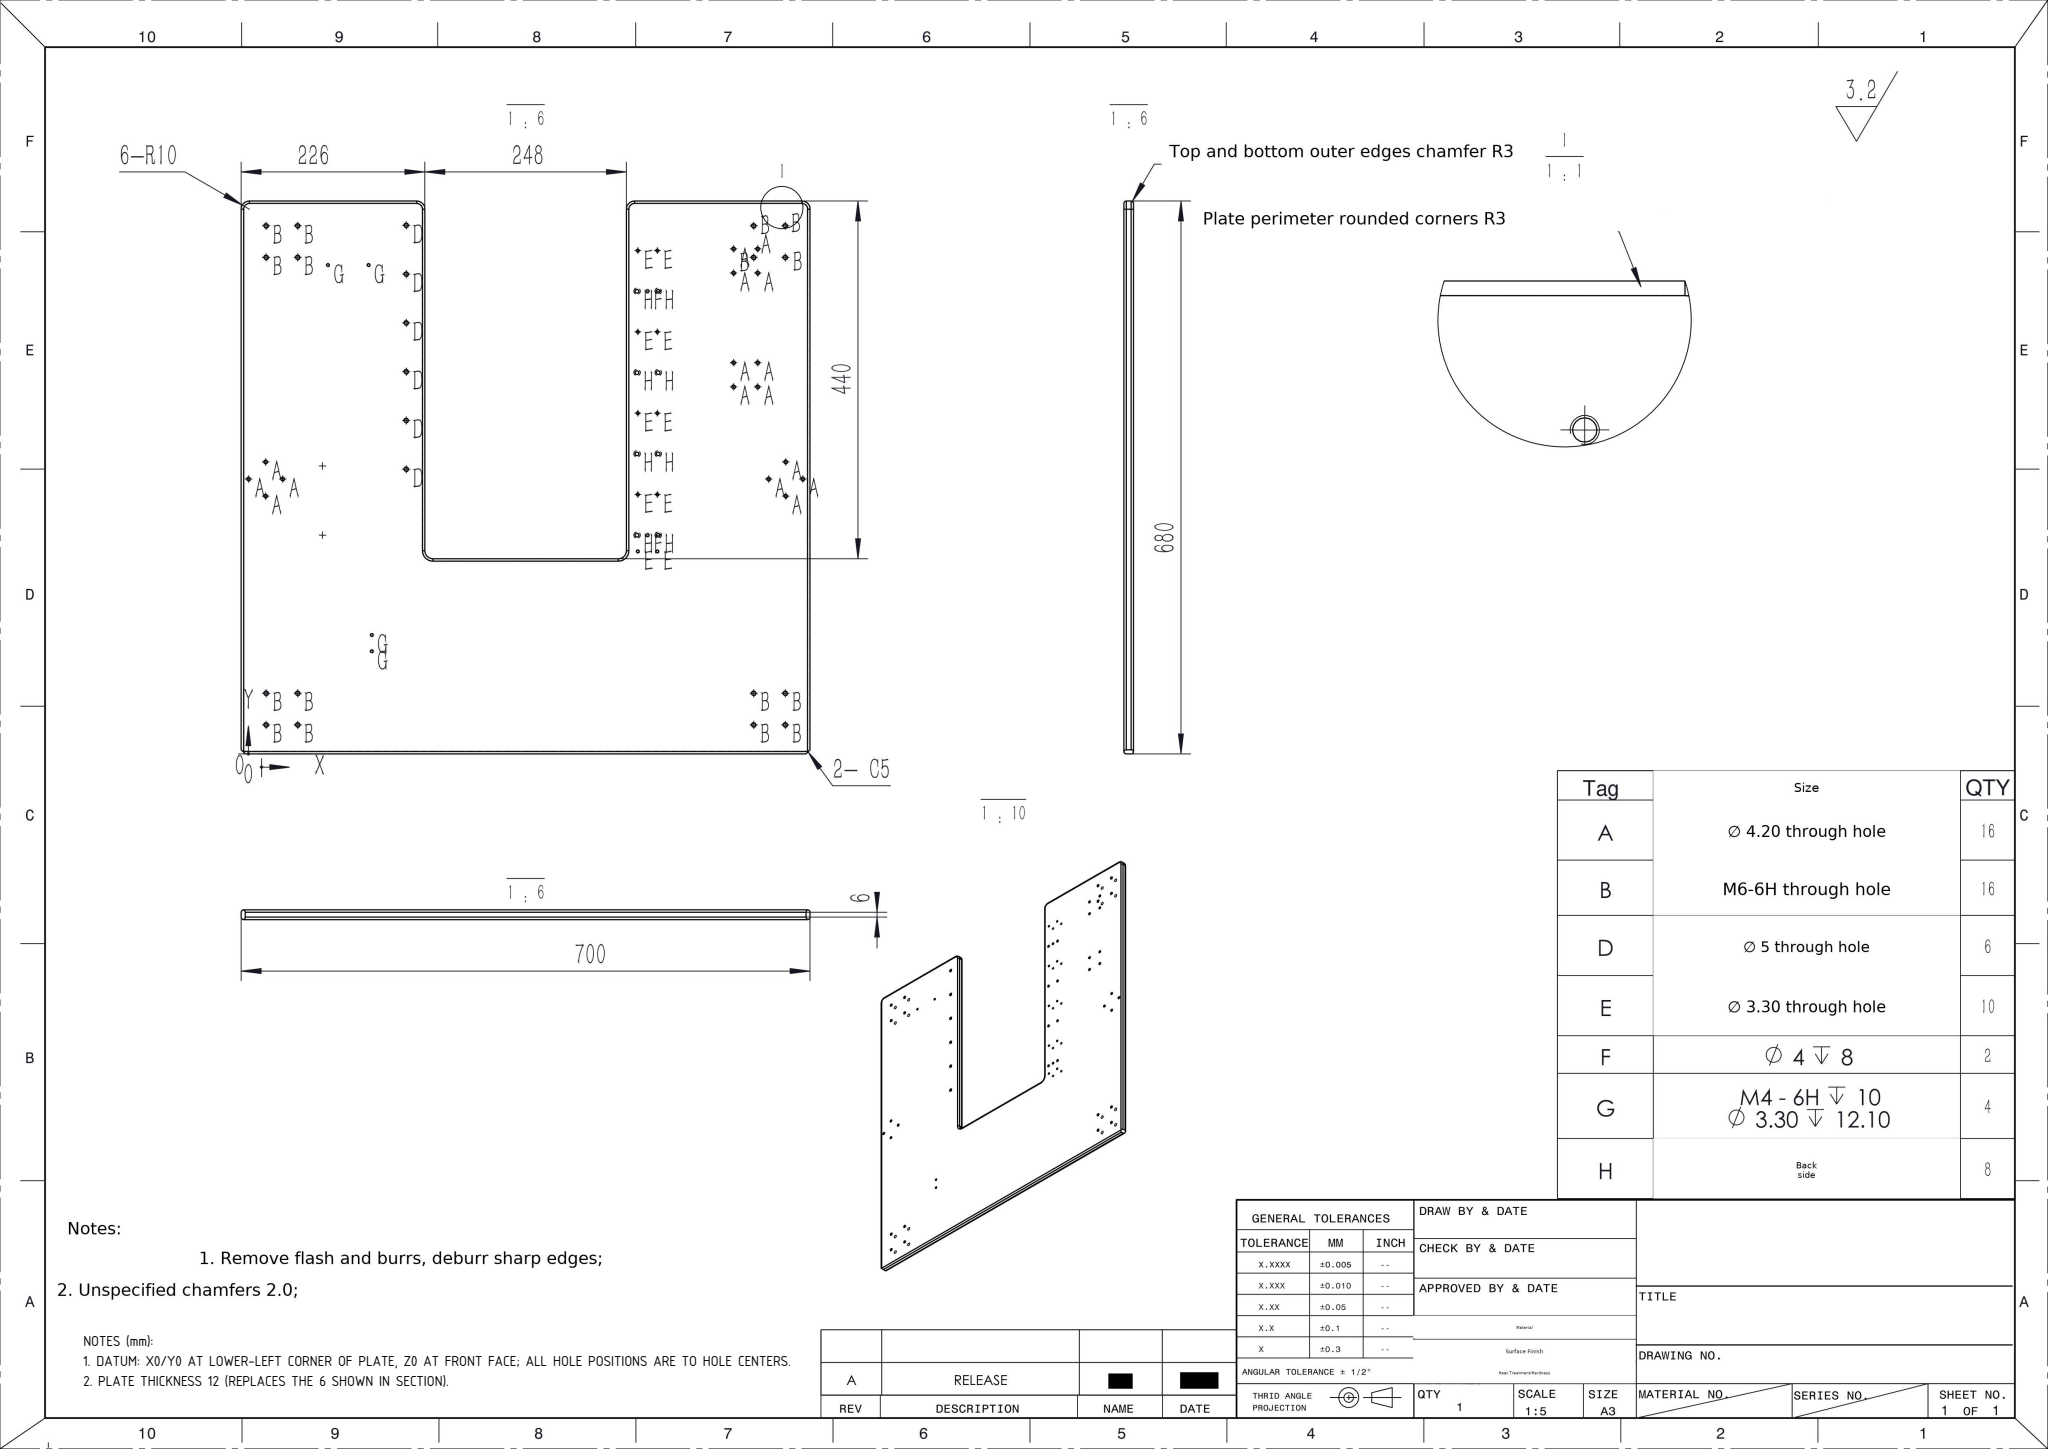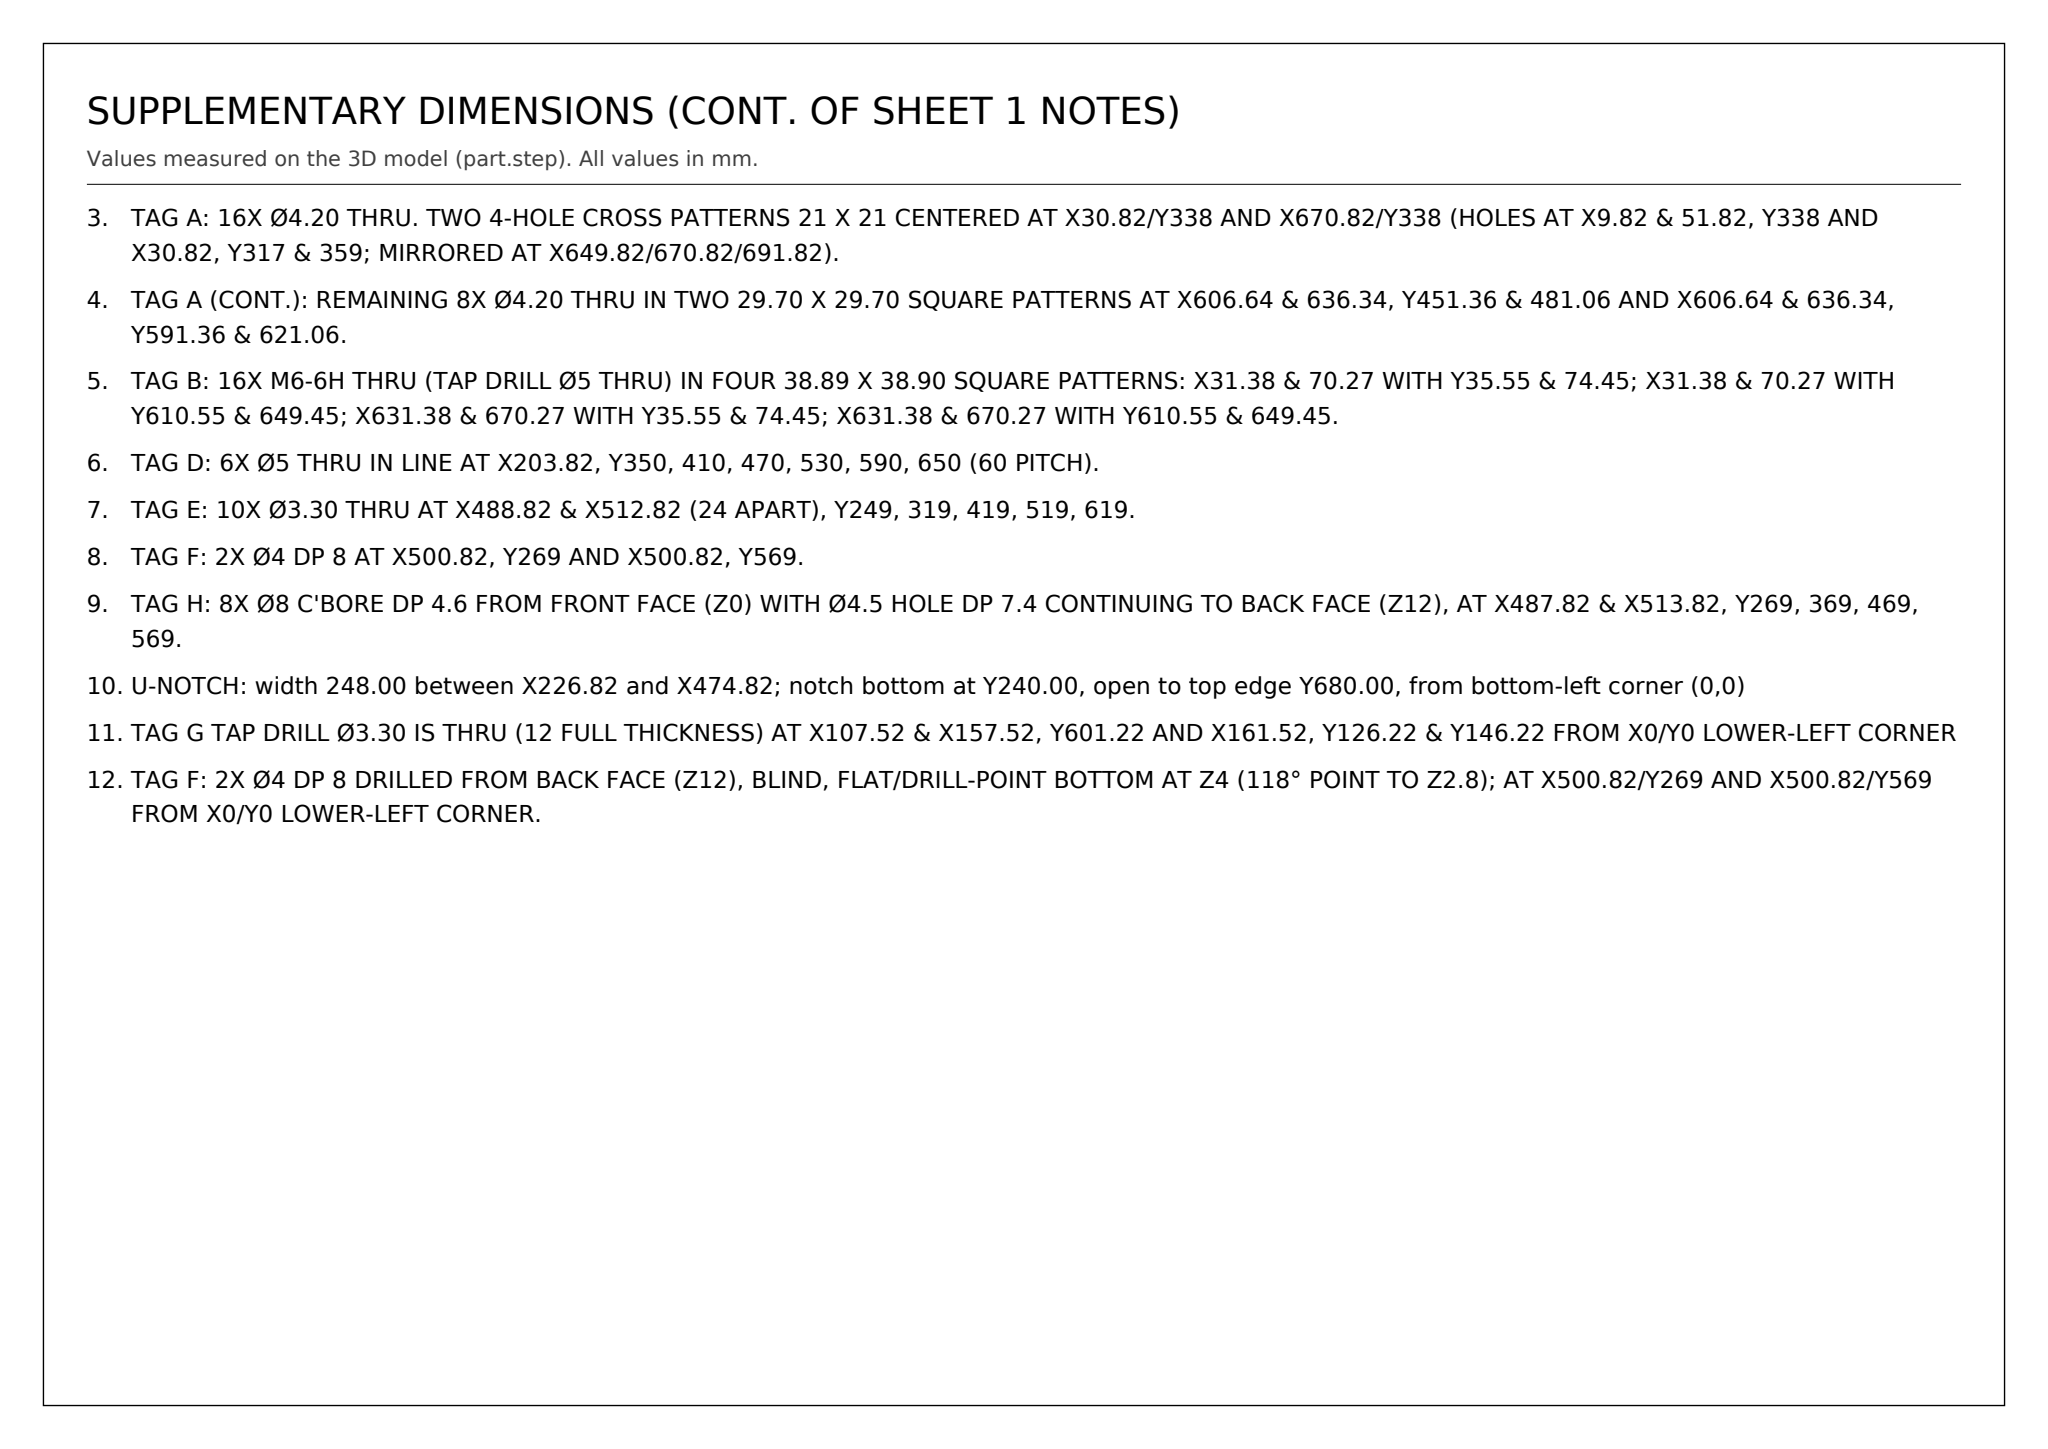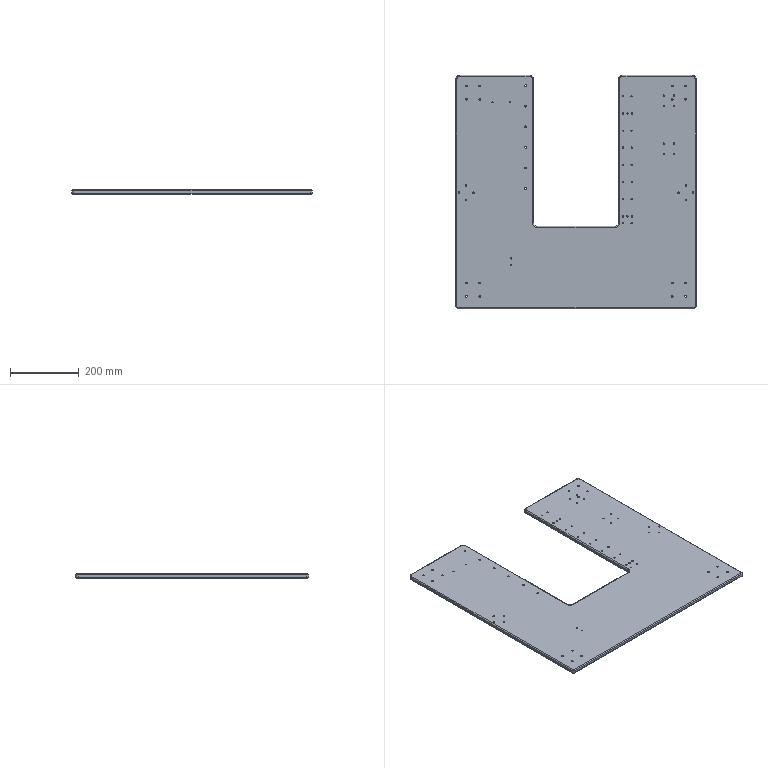Part | SolidWorks | mm | 1 solid | 198 faces | box 700 x 680 x 12 mm | volume 4375576 mm3 | cylinder 162 | plane 20 | torus 12 | cone 4 | commonest cylinder face diameters 5 x44 4.2 x32 3.3 x28 8 x16 4.5 x16 6 x16 20 x6 4 x4
Drawing notes:
DATUM: X0/Y0 AT LOWER-LEFT CORNER OF PLATE, Z0 AT FRONT FACE; ALL HOLE POSITIONS ARE TO HOLE CENTERS. | from the solid: origin_note: positions from min corner of bbox 701.648 x 680.824 x 12.0
PLATE THICKNESS 12 (REPLACES THE 6 SHOWN IN SECTION). | from the solid: bbox_xyz z = 12.0; all THRU cylinders length 12.0
TAG A: 16X Ø4.20 THRU. TWO 4-HOLE CROSS PATTERNS 21 X 21 CENTERED AT X30.82/Y338 AND X670.82/Y338 (HOLES AT X9.82 & 51.82, Y338 AND X30.82, Y317 & 359; MIRRORED AT X649.82/670.82/691.82). | from the solid: cylinders dia 4.2 z at (9.82,338),(30.82,317),(30.82,359),(51.82,338),(649.82,338),(670.82,317),(670.82,359),(691.82,338), length 12.0
TAG A (CONT.): REMAINING 8X Ø4.20 THRU IN TWO 29.70 X 29.70 SQUARE PATTERNS AT X606.64 & 636.34, Y451.36 & 481.06 AND X606.64 & 636.34, Y591.36 & 621.06. | from the solid: cylinders dia 4.2 z at (606.64/636.34, 451.36/481.06) and (606.64/636.34, 591.36/621.06), length 12.0
TAG B: 16X M6-6H THRU (TAP DRILL Ø5 THRU) IN FOUR 38.89 X 38.90 SQUARE PATTERNS: X31.38 & 70.27 WITH Y35.55 & 74.45; X31.38 & 70.27 WITH Y610.55 & 649.45; X631.38 & 670.27 WITH Y35.55 & 74.45; X631.38 & 670.27 WITH Y610.55 & 649.45. | from the solid: cylinders dia 5.0 z at x 31.38/70.27/631.38/670.27 with y 35.55/74.45/610.55/649.45, length 12.0
TAG D: 6X Ø5 THRU IN LINE AT X203.82, Y350, 410, 470, 530, 590, 650 (60 PITCH). | from the solid: cylinders dia 5.0 z at (203.82, 350/410/470/530/590/650), length 12.0
TAG E: 10X Ø3.30 THRU AT X488.82 & X512.82 (24 APART), Y249, 319, 419, 519, 619. | from the solid: cylinders dia 3.3 z at (488.82 and 512.82, y 249/319/419/519/619), length 12.0
TAG F: 2X Ø4 DP 8 AT X500.82, Y269 AND X500.82, Y569. | from the solid: cylinders dia 4.0 z at (500.82,269) and (500.82,569), length 8.0
TAG H: 8X Ø8 C'BORE DP 4.6 FROM FRONT FACE (Z0) WITH Ø4.5 HOLE DP 7.4 CONTINUING TO BACK FACE (Z12), AT X487.82 & X513.82, Y269, 369, 469, 569. | from the solid: Flat c'bore bottoms at z=4.6 over X483.8-491.8 and X509.8-517.8 with Y265-273/365-373/465-473/565-573 (8 places, 8x8 => Ø8, open at z0 front face); Ø4.5 cylinders at X487.8 & 513.8, Y269/369/469/569 run from z=4.6 to z=12.0 (7.4 deep).
U-NOTCH: width 248.00 between X226.82 and X474.82; notch bottom at Y240.00, open to top edge Y680.00, from bottom-left corner (0,0) | from the solid: axis_planes x 226.82 and 474.82; y 240.0 and y 680.0
TAG G TAP DRILL Ø3.30 IS THRU (12 FULL THICKNESS) AT X107.52 & X157.52, Y601.22 AND X161.52, Y126.22 & Y146.22 FROM X0/Y0 LOWER-LEFT CORNER | from the solid: cylinders dia 3.3 axis z length 12.0 at (107.52,601.22),(157.52,601.22),(161.52,126.22),(161.52,146.22)
TAG F: 2X Ø4 DP 8 DRILLED FROM BACK FACE (Z12), BLIND, FLAT/DRILL-POINT BOTTOM AT Z4 (118° POINT TO Z2.8); AT X500.82/Y269 AND X500.82/Y569 FROM X0/Y0 LOWER-LEFT CORNER. | from the solid: cylinders: hole/bore dia 4.0 axis z at (500.8,269.0) and (500.8,569.0) from 4.0 to 12.0 (part thickness 12, Z0 = front face); cones 118° ref dia 4.0 bbox_from z 2.8